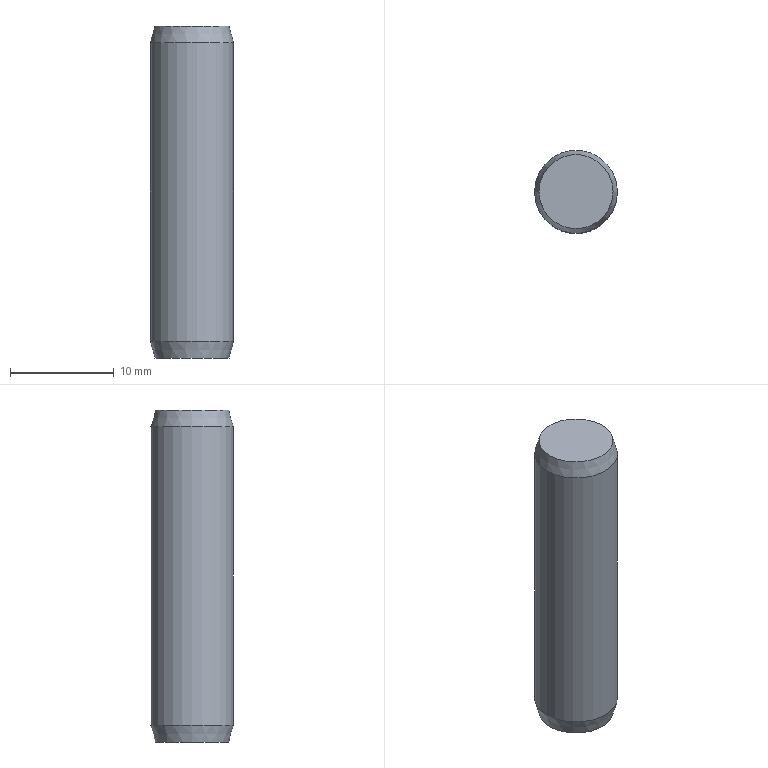Component | NX | GB-T119_1-2000_8X32 | 1 solid | 5 faces | box 8 x 8 x 32 mm | volume 1592 mm3 | plane 2 | cone 2 | cylinder 1 | commonest cylinder face diameters 8 x1
STEP:
#1=CARTESIAN_POINT('',(0.,0.,0.));
#2=DIRECTION('',(0.,0.,1.));
#3=DIRECTION('',(1.,0.,0.));
#4=AXIS2_PLACEMENT_3D('',#1,#2,#3);
#5=CARTESIAN_POINT('',(81.929,-0.,89.5));
#6=VERTEX_POINT('',#5);
#7=CARTESIAN_POINT('',(85.5,-0.,89.5));
#8=DIRECTION('',(0.,0.,-1.));
#9=DIRECTION('',(-1.,0.,0.));
#10=AXIS2_PLACEMENT_3D('',#7,#8,#9);
#11=CIRCLE('',#10,3.571);
#12=CARTESIAN_POINT('',(85.5,-0.,89.5));
#13=DIRECTION('',(0.,0.,-1.));
#14=DIRECTION('',(-1.,0.,0.));
#15=AXIS2_PLACEMENT_3D('',#12,#13,#14);
#16=PLANE('',#15);
#17=CARTESIAN_POINT('',(0.,0.));
#18=DIRECTION('',(1.,0.));
#19=AXIS2_PLACEMENT_2D('',#17,#18);
#20=CIRCLE('',#19,3.571);
#21=(GEOMETRIC_REPRESENTATION_CONTEXT(2)PARAMETRIC_REPRESENTATION_CONTEXT()REPRESENTATION_CONTEXT('',''));
#22=DEFINITIONAL_REPRESENTATION('',(#20),#21);
#23=PCURVE('',#16,#22);
#24=CARTESIAN_POINT('',(85.5,-0.,89.5));
#25=DIRECTION('',(0.,0.,1.));
#26=DIRECTION('',(1.,0.,0.));
#27=AXIS2_PLACEMENT_3D('',#24,#25,#26);
#28=CONICAL_SURFACE('',#27,3.571,0.2618);
#29=CARTESIAN_POINT('',(9.425,0.));
#30=DIRECTION('',(-1.,0.));
#31=VECTOR('',#30,1.);
#32=LINE('',#29,#31);
#33=(GEOMETRIC_REPRESENTATION_CONTEXT(2)PARAMETRIC_REPRESENTATION_CONTEXT()REPRESENTATION_CONTEXT('',''));
#34=DEFINITIONAL_REPRESENTATION('',(#32),#33);
#35=PCURVE('',#28,#34);
#36=SURFACE_CURVE('',#11,(#23,#35),.PCURVE_S1.);
#37=EDGE_CURVE('',#6,#6,#36,.T.);
#38=ORIENTED_EDGE('',*,*,#37,.T.);
#39=EDGE_LOOP('',(#38));
#40=FACE_BOUND('',#39,.T.);
#41=ADVANCED_FACE('',(#40),#16,.T.);
#42=CARTESIAN_POINT('',(81.5,-0.,91.1));
#43=VERTEX_POINT('',#42);
#44=CARTESIAN_POINT('',(85.5,-0.,91.1));
#45=DIRECTION('',(0.,0.,-1.));
#46=DIRECTION('',(-1.,0.,0.));
#47=AXIS2_PLACEMENT_3D('',#44,#45,#46);
#48=CIRCLE('',#47,4.);
#49=CARTESIAN_POINT('',(9.425,1.6));
#50=DIRECTION('',(-1.,0.));
#51=VECTOR('',#50,1.);
#52=LINE('',#49,#51);
#53=(GEOMETRIC_REPRESENTATION_CONTEXT(2)PARAMETRIC_REPRESENTATION_CONTEXT()REPRESENTATION_CONTEXT('',''));
#54=DEFINITIONAL_REPRESENTATION('',(#52),#53);
#55=PCURVE('',#28,#54);
#56=CARTESIAN_POINT('',(85.5,-0.,121.5));
#57=DIRECTION('',(0.,0.,-1.));
#58=DIRECTION('',(-1.,0.,0.));
#59=AXIS2_PLACEMENT_3D('',#56,#57,#58);
#60=CYLINDRICAL_SURFACE('',#59,4.);
#61=CARTESIAN_POINT('',(0.,30.4));
#62=DIRECTION('',(1.,0.));
#63=VECTOR('',#62,1.);
#64=LINE('',#61,#63);
#65=(GEOMETRIC_REPRESENTATION_CONTEXT(2)PARAMETRIC_REPRESENTATION_CONTEXT()REPRESENTATION_CONTEXT('',''));
#66=DEFINITIONAL_REPRESENTATION('',(#64),#65);
#67=PCURVE('',#60,#66);
#68=SURFACE_CURVE('',#48,(#55,#67),.PCURVE_S1.);
#69=EDGE_CURVE('',#43,#43,#68,.T.);
#70=ORIENTED_EDGE('',*,*,#69,.T.);
#71=CARTESIAN_POINT('',(81.929,-0.,89.5));
#72=CARTESIAN_POINT('',(81.5,-0.,91.1));
#73=B_SPLINE_CURVE_WITH_KNOTS('',1,(#71,#72),.UNSPECIFIED.,.F.,.F.,(2,2),(0.,1.656),.PIECEWISE_BEZIER_KNOTS.);
#74=CARTESIAN_POINT('',(3.142,0.));
#75=DIRECTION('',(0.,1.));
#76=VECTOR('',#75,1.);
#77=LINE('',#74,#76);
#78=(GEOMETRIC_REPRESENTATION_CONTEXT(2)PARAMETRIC_REPRESENTATION_CONTEXT()REPRESENTATION_CONTEXT('',''));
#79=DEFINITIONAL_REPRESENTATION('',(#77),#78);
#80=PCURVE('',#28,#79);
#81=CARTESIAN_POINT('',(9.425,0.));
#82=DIRECTION('',(0.,1.));
#83=VECTOR('',#82,1.);
#84=LINE('',#81,#83);
#85=(GEOMETRIC_REPRESENTATION_CONTEXT(2)PARAMETRIC_REPRESENTATION_CONTEXT()REPRESENTATION_CONTEXT('',''));
#86=DEFINITIONAL_REPRESENTATION('',(#84),#85);
#87=PCURVE('',#28,#86);
#88=SEAM_CURVE('',#73,(#80,#87),.PCURVE_S1.);
#89=EDGE_CURVE('',#6,#43,#88,.T.);
#90=ORIENTED_EDGE('',*,*,#89,.F.);
#91=ORIENTED_EDGE('',*,*,#37,.F.);
#92=ORIENTED_EDGE('',*,*,#89,.T.);
#93=EDGE_LOOP('',(#70,#90,#91,#92));
#94=FACE_BOUND('',#93,.T.);
#95=ADVANCED_FACE('',(#94),#28,.T.);
#96=CARTESIAN_POINT('',(81.5,-0.,119.9));
#97=VERTEX_POINT('',#96);
#98=CARTESIAN_POINT('',(85.5,-0.,119.9));
#99=DIRECTION('',(0.,0.,-1.));
#100=DIRECTION('',(-1.,0.,0.));
#101=AXIS2_PLACEMENT_3D('',#98,#99,#100);
#102=CIRCLE('',#101,4.);
#103=CARTESIAN_POINT('',(0.,1.6));
#104=DIRECTION('',(1.,0.));
#105=VECTOR('',#104,1.);
#106=LINE('',#103,#105);
#107=(GEOMETRIC_REPRESENTATION_CONTEXT(2)PARAMETRIC_REPRESENTATION_CONTEXT()REPRESENTATION_CONTEXT('',''));
#108=DEFINITIONAL_REPRESENTATION('',(#106),#107);
#109=PCURVE('',#60,#108);
#110=CARTESIAN_POINT('',(85.5,-0.,119.9));
#111=DIRECTION('',(0.,0.,-1.));
#112=DIRECTION('',(-1.,0.,0.));
#113=AXIS2_PLACEMENT_3D('',#110,#111,#112);
#114=CONICAL_SURFACE('',#113,4.,0.2618);
#115=CARTESIAN_POINT('',(0.,0.));
#116=DIRECTION('',(1.,0.));
#117=VECTOR('',#116,1.);
#118=LINE('',#115,#117);
#119=(GEOMETRIC_REPRESENTATION_CONTEXT(2)PARAMETRIC_REPRESENTATION_CONTEXT()REPRESENTATION_CONTEXT('',''));
#120=DEFINITIONAL_REPRESENTATION('',(#118),#119);
#121=PCURVE('',#114,#120);
#122=SURFACE_CURVE('',#102,(#109,#121),.PCURVE_S1.);
#123=EDGE_CURVE('',#97,#97,#122,.T.);
#124=ORIENTED_EDGE('',*,*,#123,.T.);
#125=CARTESIAN_POINT('',(81.5,-0.,119.9));
#126=CARTESIAN_POINT('',(81.5,-0.,91.1));
#127=B_SPLINE_CURVE_WITH_KNOTS('',1,(#125,#126),.UNSPECIFIED.,.F.,.F.,(2,2),(1.6,30.4),.PIECEWISE_BEZIER_KNOTS.);
#128=CARTESIAN_POINT('',(6.283,0.));
#129=DIRECTION('',(0.,1.));
#130=VECTOR('',#129,1.);
#131=LINE('',#128,#130);
#132=(GEOMETRIC_REPRESENTATION_CONTEXT(2)PARAMETRIC_REPRESENTATION_CONTEXT()REPRESENTATION_CONTEXT('',''));
#133=DEFINITIONAL_REPRESENTATION('',(#131),#132);
#134=PCURVE('',#60,#133);
#135=CARTESIAN_POINT('',(0.,0.));
#136=DIRECTION('',(0.,1.));
#137=VECTOR('',#136,1.);
#138=LINE('',#135,#137);
#139=(GEOMETRIC_REPRESENTATION_CONTEXT(2)PARAMETRIC_REPRESENTATION_CONTEXT()REPRESENTATION_CONTEXT('',''));
#140=DEFINITIONAL_REPRESENTATION('',(#138),#139);
#141=PCURVE('',#60,#140);
#142=SEAM_CURVE('',#127,(#134,#141),.PCURVE_S1.);
#143=EDGE_CURVE('',#97,#43,#142,.T.);
#144=ORIENTED_EDGE('',*,*,#143,.T.);
#145=ORIENTED_EDGE('',*,*,#69,.F.);
#146=ORIENTED_EDGE('',*,*,#143,.F.);
#147=EDGE_LOOP('',(#124,#144,#145,#146));
#148=FACE_BOUND('',#147,.T.);
#149=ADVANCED_FACE('',(#148),#60,.T.);
#150=CARTESIAN_POINT('',(81.929,-0.,121.5));
#151=VERTEX_POINT('',#150);
#152=CARTESIAN_POINT('',(85.5,-0.,121.5));
#153=DIRECTION('',(0.,0.,-1.));
#154=DIRECTION('',(-1.,0.,0.));
#155=AXIS2_PLACEMENT_3D('',#152,#153,#154);
#156=CIRCLE('',#155,3.571);
#157=CARTESIAN_POINT('',(0.,-1.6));
#158=DIRECTION('',(1.,0.));
#159=VECTOR('',#158,1.);
#160=LINE('',#157,#159);
#161=(GEOMETRIC_REPRESENTATION_CONTEXT(2)PARAMETRIC_REPRESENTATION_CONTEXT()REPRESENTATION_CONTEXT('',''));
#162=DEFINITIONAL_REPRESENTATION('',(#160),#161);
#163=PCURVE('',#114,#162);
#164=CARTESIAN_POINT('',(89.071,-0.,121.5));
#165=DIRECTION('',(0.,0.,1.));
#166=DIRECTION('',(1.,0.,0.));
#167=AXIS2_PLACEMENT_3D('',#164,#165,#166);
#168=PLANE('',#167);
#169=CARTESIAN_POINT('',(-7.143,0.));
#170=CARTESIAN_POINT('',(-7.143,6.186));
#171=CARTESIAN_POINT('',(-1.786,3.093));
#172=CARTESIAN_POINT('',(3.571,0.));
#173=CARTESIAN_POINT('',(-1.786,-3.093));
#174=CARTESIAN_POINT('',(-7.143,-6.186));
#175=CARTESIAN_POINT('',(-7.143,0.));
#176=(BOUNDED_CURVE()B_SPLINE_CURVE(2,(#169,#170,#171,#172,#173,#174,#175),.UNSPECIFIED.,.T.,.F.)B_SPLINE_CURVE_WITH_KNOTS((1,2,2,2,2,1),(-2.094,0.,2.094,4.189,6.283,8.378),.UNSPECIFIED.)CURVE()GEOMETRIC_REPRESENTATION_ITEM()RATIONAL_B_SPLINE_CURVE((1.,0.5,1.,0.5,1.,0.5,1.))REPRESENTATION_ITEM(''));
#177=(GEOMETRIC_REPRESENTATION_CONTEXT(2)PARAMETRIC_REPRESENTATION_CONTEXT()REPRESENTATION_CONTEXT('',''));
#178=DEFINITIONAL_REPRESENTATION('',(#176),#177);
#179=PCURVE('',#168,#178);
#180=SURFACE_CURVE('',#156,(#163,#179),.PCURVE_S1.);
#181=EDGE_CURVE('',#151,#151,#180,.T.);
#182=ORIENTED_EDGE('',*,*,#181,.T.);
#183=CARTESIAN_POINT('',(81.929,-0.,121.5));
#184=CARTESIAN_POINT('',(81.5,-0.,119.9));
#185=B_SPLINE_CURVE_WITH_KNOTS('',1,(#183,#184),.UNSPECIFIED.,.F.,.F.,(2,2),(-1.656,0.),.PIECEWISE_BEZIER_KNOTS.);
#186=CARTESIAN_POINT('',(6.283,0.));
#187=DIRECTION('',(0.,1.));
#188=VECTOR('',#187,1.);
#189=LINE('',#186,#188);
#190=(GEOMETRIC_REPRESENTATION_CONTEXT(2)PARAMETRIC_REPRESENTATION_CONTEXT()REPRESENTATION_CONTEXT('',''));
#191=DEFINITIONAL_REPRESENTATION('',(#189),#190);
#192=PCURVE('',#114,#191);
#193=CARTESIAN_POINT('',(0.,0.));
#194=DIRECTION('',(0.,1.));
#195=VECTOR('',#194,1.);
#196=LINE('',#193,#195);
#197=(GEOMETRIC_REPRESENTATION_CONTEXT(2)PARAMETRIC_REPRESENTATION_CONTEXT()REPRESENTATION_CONTEXT('',''));
#198=DEFINITIONAL_REPRESENTATION('',(#196),#197);
#199=PCURVE('',#114,#198);
#200=SEAM_CURVE('',#185,(#192,#199),.PCURVE_S1.);
#201=EDGE_CURVE('',#151,#97,#200,.T.);
#202=ORIENTED_EDGE('',*,*,#201,.T.);
#203=ORIENTED_EDGE('',*,*,#123,.F.);
#204=ORIENTED_EDGE('',*,*,#201,.F.);
#205=EDGE_LOOP('',(#182,#202,#203,#204));
#206=FACE_BOUND('',#205,.T.);
#207=ADVANCED_FACE('',(#206),#114,.T.);
#208=ORIENTED_EDGE('',*,*,#181,.F.);
#209=EDGE_LOOP('',(#208));
#210=FACE_BOUND('',#209,.T.);
#211=ADVANCED_FACE('',(#210),#168,.T.);
#212=CLOSED_SHELL('',(#41,#95,#149,#207,#211));
#213=MANIFOLD_SOLID_BREP('',#212);
#214=(LENGTH_UNIT()NAMED_UNIT(*)SI_UNIT(.MILLI.,.METRE.));
#215=UNCERTAINTY_MEASURE_WITH_UNIT(LENGTH_MEASURE(0.00001),#214,'','');
#216=(NAMED_UNIT(*)PLANE_ANGLE_UNIT()SI_UNIT($,.RADIAN.));
#217=(NAMED_UNIT(*)SI_UNIT($,.STERADIAN.)SOLID_ANGLE_UNIT());
#218=(GEOMETRIC_REPRESENTATION_CONTEXT(3)GLOBAL_UNCERTAINTY_ASSIGNED_CONTEXT((#215))GLOBAL_UNIT_ASSIGNED_CONTEXT((#214,#216,#217))REPRESENTATION_CONTEXT('',''));
#219=ADVANCED_BREP_SHAPE_REPRESENTATION('',(#4,#213),#218);